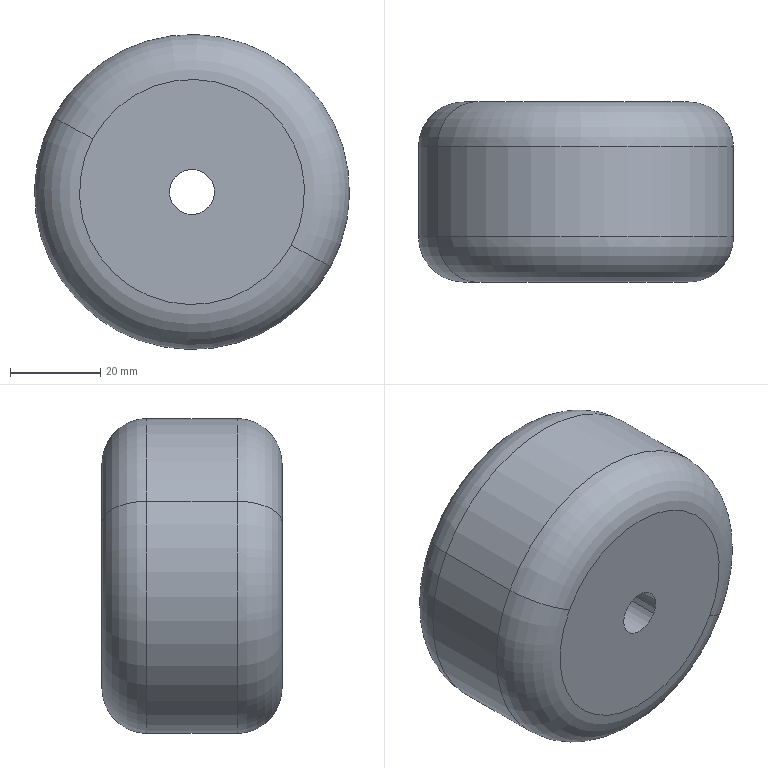Component | SolidWorks | AssemblyVibratoryFeederChassis-1_AssemblyWheel-1_Wheel-1 | 1 solid | 10 faces | box 70 x 40 x 70 mm | volume 141960 mm3 | torus 4 | cylinder 4 | plane 2 | commonest cylinder face diameters 10 x2 70 x2
build123d program:
from build123d import *

# Parameters (mm, degrees)
SKETCH1_R      = 35
SKETCH1_R_2    = 5
EXTRUDE1_DEPTH = 40
FILLET1_R      = 10


with BuildPart() as part:
    # Sketch1 → Extrude1 (new body)
    with BuildSketch(Plane.XY):
        Circle(SKETCH1_R)
        Circle(SKETCH1_R_2, mode=Mode.SUBTRACT)
    extrude(amount=-EXTRUDE1_DEPTH)

    # Fillet1
    fillet1_edges = [part.edges().sort_by_distance(p)[0] for p in [
        (-35, 0, 0),
        (-35, 0, -40),
    ]]
    fillet(fillet1_edges, radius=FILLET1_R)


solid = part.part

# Placed as in the assembly
solid = solid.moved(Location((-277.449, -301.176, -142.722), (90, 0, 0)))
STEP:
#1=COLOUR_RGB('',0.7922,0.8196,0.9333);
#2=FILL_AREA_STYLE_COLOUR('',#1);
#3=FILL_AREA_STYLE('',(#2));
#4=SURFACE_STYLE_FILL_AREA(#3);
#5=SURFACE_SIDE_STYLE('',(#4));
#6=SURFACE_STYLE_USAGE(.BOTH.,#5);
#7=PRESENTATION_STYLE_ASSIGNMENT((#6));
#8=CARTESIAN_POINT('',(-12.137,-11.464,-4.966));
#9=VERTEX_POINT('',#8);
#10=CARTESIAN_POINT('',(-9.71,-11.464,-6.272));
#11=VERTEX_POINT('',#10);
#12=CARTESIAN_POINT('',(-10.923,-11.464,-5.619));
#13=DIRECTION('',(0.,1.,-0.));
#14=DIRECTION('',(0.8806,0.,-0.4738));
#15=AXIS2_PLACEMENT_3D('',#12,#13,#14);
#16=CIRCLE('',#15,1.378);
#17=EDGE_CURVE('',#9,#11,#16,.T.);
#18=ORIENTED_EDGE('',*,*,#17,.F.);
#19=CARTESIAN_POINT('',(-11.79,-11.857,-5.153));
#20=VERTEX_POINT('',#19);
#21=CARTESIAN_POINT('',(-11.79,-11.464,-5.153));
#22=DIRECTION('',(0.4738,0.,0.8806));
#23=DIRECTION('',(0.8806,0.,-0.4738));
#24=AXIS2_PLACEMENT_3D('',#21,#22,#23);
#25=CIRCLE('',#24,0.3937);
#26=EDGE_CURVE('',#9,#20,#25,.T.);
#27=ORIENTED_EDGE('',*,*,#26,.T.);
#28=CARTESIAN_POINT('',(-10.056,-11.857,-6.085));
#29=VERTEX_POINT('',#28);
#30=CARTESIAN_POINT('',(-10.923,-11.857,-5.619));
#31=DIRECTION('',(-0.,-1.,0.));
#32=DIRECTION('',(0.8806,0.,-0.4738));
#33=AXIS2_PLACEMENT_3D('',#30,#31,#32);
#34=CIRCLE('',#33,0.9843);
#35=EDGE_CURVE('',#29,#20,#34,.T.);
#36=ORIENTED_EDGE('',*,*,#35,.F.);
#37=CARTESIAN_POINT('',(-10.056,-11.464,-6.085));
#38=DIRECTION('',(-0.4738,-0.,-0.8806));
#39=DIRECTION('',(-0.8806,0.,0.4738));
#40=AXIS2_PLACEMENT_3D('',#37,#38,#39);
#41=CIRCLE('',#40,0.3937);
#42=EDGE_CURVE('',#11,#29,#41,.T.);
#43=ORIENTED_EDGE('',*,*,#42,.F.);
#44=EDGE_LOOP('',(#18,#27,#36,#43));
#45=FACE_OUTER_BOUND('',#44,.T.);
#46=CARTESIAN_POINT('',(-10.923,-11.464,-5.619));
#47=DIRECTION('',(-0.,-1.,0.));
#48=DIRECTION('',(0.8806,-0.,-0.4738));
#49=AXIS2_PLACEMENT_3D('',#46,#47,#48);
#50=TOROIDAL_SURFACE('',#49,0.9843,0.3937);
#51=ADVANCED_FACE('',(#45),#50,.T.);
#52=CARTESIAN_POINT('',(-11.79,-10.283,-5.153));
#53=VERTEX_POINT('',#52);
#54=CARTESIAN_POINT('',(-10.056,-10.283,-6.085));
#55=VERTEX_POINT('',#54);
#56=CARTESIAN_POINT('',(-10.923,-10.283,-5.619));
#57=DIRECTION('',(0.,1.,-0.));
#58=DIRECTION('',(0.8806,0.,-0.4738));
#59=AXIS2_PLACEMENT_3D('',#56,#57,#58);
#60=CIRCLE('',#59,0.9843);
#61=EDGE_CURVE('',#53,#55,#60,.T.);
#62=ORIENTED_EDGE('',*,*,#61,.F.);
#63=CARTESIAN_POINT('',(-12.137,-10.676,-4.966));
#64=VERTEX_POINT('',#63);
#65=CARTESIAN_POINT('',(-11.79,-10.676,-5.153));
#66=DIRECTION('',(0.4738,0.,0.8806));
#67=DIRECTION('',(0.8806,0.,-0.4738));
#68=AXIS2_PLACEMENT_3D('',#65,#66,#67);
#69=CIRCLE('',#68,0.3937);
#70=EDGE_CURVE('',#53,#64,#69,.T.);
#71=ORIENTED_EDGE('',*,*,#70,.T.);
#72=CARTESIAN_POINT('',(-9.71,-10.676,-6.272));
#73=VERTEX_POINT('',#72);
#74=CARTESIAN_POINT('',(-10.923,-10.676,-5.619));
#75=DIRECTION('',(-0.,-1.,0.));
#76=DIRECTION('',(0.8806,0.,-0.4738));
#77=AXIS2_PLACEMENT_3D('',#74,#75,#76);
#78=CIRCLE('',#77,1.378);
#79=EDGE_CURVE('',#73,#64,#78,.T.);
#80=ORIENTED_EDGE('',*,*,#79,.F.);
#81=CARTESIAN_POINT('',(-10.056,-10.676,-6.085));
#82=DIRECTION('',(-0.4738,-0.,-0.8806));
#83=DIRECTION('',(-0.8806,0.,0.4738));
#84=AXIS2_PLACEMENT_3D('',#81,#82,#83);
#85=CIRCLE('',#84,0.3937);
#86=EDGE_CURVE('',#55,#73,#85,.T.);
#87=ORIENTED_EDGE('',*,*,#86,.F.);
#88=EDGE_LOOP('',(#62,#71,#80,#87));
#89=FACE_OUTER_BOUND('',#88,.T.);
#90=CARTESIAN_POINT('',(-10.923,-10.676,-5.619));
#91=DIRECTION('',(-0.,-1.,0.));
#92=DIRECTION('',(0.8806,-0.,-0.4738));
#93=AXIS2_PLACEMENT_3D('',#90,#91,#92);
#94=TOROIDAL_SURFACE('',#93,0.9843,0.3937);
#95=ADVANCED_FACE('',(#89),#94,.T.);
#96=CARTESIAN_POINT('',(-11.097,-10.283,-5.526));
#97=VERTEX_POINT('',#96);
#98=CARTESIAN_POINT('',(-10.75,-10.283,-5.712));
#99=VERTEX_POINT('',#98);
#100=CARTESIAN_POINT('',(-10.923,-10.283,-5.619));
#101=DIRECTION('',(-0.,-1.,0.));
#102=DIRECTION('',(0.8806,0.,-0.4738));
#103=AXIS2_PLACEMENT_3D('',#100,#101,#102);
#104=CIRCLE('',#103,0.1969);
#105=EDGE_CURVE('',#97,#99,#104,.T.);
#106=ORIENTED_EDGE('',*,*,#105,.F.);
#107=CARTESIAN_POINT('',(-11.097,-11.857,-5.526));
#108=VERTEX_POINT('',#107);
#109=CARTESIAN_POINT('',(-11.097,-10.283,-5.526));
#110=DIRECTION('',(-0.,-1.,0.));
#111=VECTOR('',#110,39.37);
#112=LINE('',#109,#111);
#113=EDGE_CURVE('',#97,#108,#112,.T.);
#114=ORIENTED_EDGE('',*,*,#113,.T.);
#115=CARTESIAN_POINT('',(-10.75,-11.857,-5.712));
#116=VERTEX_POINT('',#115);
#117=CARTESIAN_POINT('',(-10.923,-11.857,-5.619));
#118=DIRECTION('',(-0.,-1.,0.));
#119=DIRECTION('',(0.8806,0.,-0.4738));
#120=AXIS2_PLACEMENT_3D('',#117,#118,#119);
#121=CIRCLE('',#120,0.1969);
#122=EDGE_CURVE('',#108,#116,#121,.T.);
#123=ORIENTED_EDGE('',*,*,#122,.T.);
#124=CARTESIAN_POINT('',(-10.75,-10.283,-5.712));
#125=DIRECTION('',(-0.,-1.,0.));
#126=VECTOR('',#125,39.37);
#127=LINE('',#124,#126);
#128=EDGE_CURVE('',#99,#116,#127,.T.);
#129=ORIENTED_EDGE('',*,*,#128,.F.);
#130=EDGE_LOOP('',(#106,#114,#123,#129));
#131=FACE_OUTER_BOUND('',#130,.T.);
#132=CARTESIAN_POINT('',(-10.923,-10.283,-5.619));
#133=DIRECTION('',(-0.,-1.,0.));
#134=DIRECTION('',(0.8806,0.,-0.4738));
#135=AXIS2_PLACEMENT_3D('',#132,#133,#134);
#136=CYLINDRICAL_SURFACE('',#135,0.1969);
#137=ADVANCED_FACE('',(#131),#136,.F.);
#138=ORIENTED_EDGE('',*,*,#79,.T.);
#139=CARTESIAN_POINT('',(-12.137,-10.283,-4.966));
#140=DIRECTION('',(-0.,-1.,0.));
#141=VECTOR('',#140,39.37);
#142=LINE('',#139,#141);
#143=EDGE_CURVE('',#64,#9,#142,.T.);
#144=ORIENTED_EDGE('',*,*,#143,.T.);
#145=ORIENTED_EDGE('',*,*,#17,.T.);
#146=CARTESIAN_POINT('',(-9.71,-10.283,-6.272));
#147=DIRECTION('',(-0.,-1.,0.));
#148=VECTOR('',#147,39.37);
#149=LINE('',#146,#148);
#150=EDGE_CURVE('',#73,#11,#149,.T.);
#151=ORIENTED_EDGE('',*,*,#150,.F.);
#152=EDGE_LOOP('',(#138,#144,#145,#151));
#153=FACE_OUTER_BOUND('',#152,.T.);
#154=CARTESIAN_POINT('',(-10.923,-10.283,-5.619));
#155=DIRECTION('',(-0.,-1.,0.));
#156=DIRECTION('',(0.8806,0.,-0.4738));
#157=AXIS2_PLACEMENT_3D('',#154,#155,#156);
#158=CYLINDRICAL_SURFACE('',#157,1.378);
#159=ADVANCED_FACE('',(#153),#158,.T.);
#160=ORIENTED_EDGE('',*,*,#143,.F.);
#161=CARTESIAN_POINT('',(-10.923,-10.676,-5.619));
#162=DIRECTION('',(-0.,-1.,0.));
#163=DIRECTION('',(0.8806,0.,-0.4738));
#164=AXIS2_PLACEMENT_3D('',#161,#162,#163);
#165=CIRCLE('',#164,1.378);
#166=EDGE_CURVE('',#64,#73,#165,.T.);
#167=ORIENTED_EDGE('',*,*,#166,.T.);
#168=ORIENTED_EDGE('',*,*,#150,.T.);
#169=CARTESIAN_POINT('',(-10.923,-11.464,-5.619));
#170=DIRECTION('',(0.,1.,-0.));
#171=DIRECTION('',(0.8806,0.,-0.4738));
#172=AXIS2_PLACEMENT_3D('',#169,#170,#171);
#173=CIRCLE('',#172,1.378);
#174=EDGE_CURVE('',#11,#9,#173,.T.);
#175=ORIENTED_EDGE('',*,*,#174,.T.);
#176=EDGE_LOOP('',(#160,#167,#168,#175));
#177=FACE_OUTER_BOUND('',#176,.T.);
#178=CARTESIAN_POINT('',(-10.923,-10.283,-5.619));
#179=DIRECTION('',(-0.,-1.,0.));
#180=DIRECTION('',(0.8806,0.,-0.4738));
#181=AXIS2_PLACEMENT_3D('',#178,#179,#180);
#182=CYLINDRICAL_SURFACE('',#181,1.378);
#183=ADVANCED_FACE('',(#177),#182,.T.);
#184=CARTESIAN_POINT('',(-10.923,-10.283,-5.619));
#185=DIRECTION('',(0.,1.,-0.));
#186=DIRECTION('',(0.8806,0.,-0.4738));
#187=AXIS2_PLACEMENT_3D('',#184,#185,#186);
#188=CIRCLE('',#187,0.9843);
#189=EDGE_CURVE('',#55,#53,#188,.T.);
#190=ORIENTED_EDGE('',*,*,#189,.T.);
#191=ORIENTED_EDGE('',*,*,#61,.T.);
#192=EDGE_LOOP('',(#190,#191));
#193=FACE_OUTER_BOUND('',#192,.T.);
#194=CARTESIAN_POINT('',(-10.923,-10.283,-5.619));
#195=DIRECTION('',(-0.,-1.,0.));
#196=DIRECTION('',(0.8806,0.,-0.4738));
#197=AXIS2_PLACEMENT_3D('',#194,#195,#196);
#198=CIRCLE('',#197,0.1969);
#199=EDGE_CURVE('',#99,#97,#198,.T.);
#200=ORIENTED_EDGE('',*,*,#199,.T.);
#201=ORIENTED_EDGE('',*,*,#105,.T.);
#202=EDGE_LOOP('',(#200,#201));
#203=FACE_BOUND('',#202,.T.);
#204=CARTESIAN_POINT('',(-10.923,-10.283,-5.619));
#205=DIRECTION('',(-0.,-1.,0.));
#206=DIRECTION('',(0.8806,-0.,-0.4738));
#207=AXIS2_PLACEMENT_3D('',#204,#205,#206);
#208=PLANE('',#207);
#209=ADVANCED_FACE('',(#193,#203),#208,.F.);
#210=ORIENTED_EDGE('',*,*,#35,.T.);
#211=CARTESIAN_POINT('',(-10.923,-11.857,-5.619));
#212=DIRECTION('',(-0.,-1.,0.));
#213=DIRECTION('',(0.8806,0.,-0.4738));
#214=AXIS2_PLACEMENT_3D('',#211,#212,#213);
#215=CIRCLE('',#214,0.9843);
#216=EDGE_CURVE('',#20,#29,#215,.T.);
#217=ORIENTED_EDGE('',*,*,#216,.T.);
#218=EDGE_LOOP('',(#210,#217));
#219=FACE_OUTER_BOUND('',#218,.T.);
#220=CARTESIAN_POINT('',(-10.923,-11.857,-5.619));
#221=DIRECTION('',(-0.,-1.,0.));
#222=DIRECTION('',(0.8806,0.,-0.4738));
#223=AXIS2_PLACEMENT_3D('',#220,#221,#222);
#224=CIRCLE('',#223,0.1969);
#225=EDGE_CURVE('',#116,#108,#224,.T.);
#226=ORIENTED_EDGE('',*,*,#225,.F.);
#227=ORIENTED_EDGE('',*,*,#122,.F.);
#228=EDGE_LOOP('',(#226,#227));
#229=FACE_BOUND('',#228,.T.);
#230=CARTESIAN_POINT('',(-10.923,-11.857,-5.619));
#231=DIRECTION('',(-0.,-1.,0.));
#232=DIRECTION('',(0.8806,-0.,-0.4738));
#233=AXIS2_PLACEMENT_3D('',#230,#231,#232);
#234=PLANE('',#233);
#235=ADVANCED_FACE('',(#219,#229),#234,.T.);
#236=ORIENTED_EDGE('',*,*,#113,.F.);
#237=ORIENTED_EDGE('',*,*,#199,.F.);
#238=ORIENTED_EDGE('',*,*,#128,.T.);
#239=ORIENTED_EDGE('',*,*,#225,.T.);
#240=EDGE_LOOP('',(#236,#237,#238,#239));
#241=FACE_OUTER_BOUND('',#240,.T.);
#242=CARTESIAN_POINT('',(-10.923,-10.283,-5.619));
#243=DIRECTION('',(-0.,-1.,0.));
#244=DIRECTION('',(0.8806,0.,-0.4738));
#245=AXIS2_PLACEMENT_3D('',#242,#243,#244);
#246=CYLINDRICAL_SURFACE('',#245,0.1969);
#247=ADVANCED_FACE('',(#241),#246,.F.);
#248=ORIENTED_EDGE('',*,*,#70,.F.);
#249=ORIENTED_EDGE('',*,*,#189,.F.);
#250=ORIENTED_EDGE('',*,*,#86,.T.);
#251=ORIENTED_EDGE('',*,*,#166,.F.);
#252=EDGE_LOOP('',(#248,#249,#250,#251));
#253=FACE_OUTER_BOUND('',#252,.T.);
#254=CARTESIAN_POINT('',(-10.923,-10.676,-5.619));
#255=DIRECTION('',(-0.,-1.,0.));
#256=DIRECTION('',(0.8806,-0.,-0.4738));
#257=AXIS2_PLACEMENT_3D('',#254,#255,#256);
#258=TOROIDAL_SURFACE('',#257,0.9843,0.3937);
#259=ADVANCED_FACE('',(#253),#258,.T.);
#260=ORIENTED_EDGE('',*,*,#26,.F.);
#261=ORIENTED_EDGE('',*,*,#174,.F.);
#262=ORIENTED_EDGE('',*,*,#42,.T.);
#263=ORIENTED_EDGE('',*,*,#216,.F.);
#264=EDGE_LOOP('',(#260,#261,#262,#263));
#265=FACE_OUTER_BOUND('',#264,.T.);
#266=CARTESIAN_POINT('',(-10.923,-11.464,-5.619));
#267=DIRECTION('',(-0.,-1.,0.));
#268=DIRECTION('',(0.8806,-0.,-0.4738));
#269=AXIS2_PLACEMENT_3D('',#266,#267,#268);
#270=TOROIDAL_SURFACE('',#269,0.9843,0.3937);
#271=ADVANCED_FACE('',(#265),#270,.T.);
#272=CLOSED_SHELL('',(#51,#95,#137,#159,#183,#209,#235,#247,#259,#271));
#273=MANIFOLD_SOLID_BREP('',#272);
#274=STYLED_ITEM('',(#7),#273);
#275=(LENGTH_UNIT()NAMED_UNIT(*)SI_UNIT($,.METRE.));
#276=LENGTH_MEASURE_WITH_UNIT(LENGTH_MEASURE(0.0254),#275);
#277=DIMENSIONAL_EXPONENTS(1.,0.,0.,0.,0.,0.,0.);
#278=(CONVERSION_BASED_UNIT('',#276)LENGTH_UNIT()NAMED_UNIT(#277));
#279=UNCERTAINTY_MEASURE_WITH_UNIT(LENGTH_MEASURE(0.00001),#278,'','');
#280=(NAMED_UNIT(*)PLANE_ANGLE_UNIT()SI_UNIT($,.RADIAN.));
#281=(NAMED_UNIT(*)SI_UNIT($,.STERADIAN.)SOLID_ANGLE_UNIT());
#282=(GEOMETRIC_REPRESENTATION_CONTEXT(3)GLOBAL_UNCERTAINTY_ASSIGNED_CONTEXT((#279))GLOBAL_UNIT_ASSIGNED_CONTEXT((#278,#280,#281))REPRESENTATION_CONTEXT('',''));
#283=MECHANICAL_DESIGN_GEOMETRIC_PRESENTATION_REPRESENTATION('',(#274),#282);
#284=PRESENTATION_LAYER_ASSIGNMENT('','',(#274));
#285=CARTESIAN_POINT('',(0.,0.,0.));
#286=DIRECTION('',(0.,0.,1.));
#287=DIRECTION('',(1.,0.,0.));
#288=AXIS2_PLACEMENT_3D('',#285,#286,#287);
#289=(LENGTH_UNIT()NAMED_UNIT(*)SI_UNIT($,.METRE.));
#290=LENGTH_MEASURE_WITH_UNIT(LENGTH_MEASURE(0.0254),#289);
#291=DIMENSIONAL_EXPONENTS(1.,0.,0.,0.,0.,0.,0.);
#292=(CONVERSION_BASED_UNIT('',#290)LENGTH_UNIT()NAMED_UNIT(#291));
#293=UNCERTAINTY_MEASURE_WITH_UNIT(LENGTH_MEASURE(0.00001),#292,'','');
#294=(NAMED_UNIT(*)PLANE_ANGLE_UNIT()SI_UNIT($,.RADIAN.));
#295=(NAMED_UNIT(*)SI_UNIT($,.STERADIAN.)SOLID_ANGLE_UNIT());
#296=(GEOMETRIC_REPRESENTATION_CONTEXT(3)GLOBAL_UNCERTAINTY_ASSIGNED_CONTEXT((#293))GLOBAL_UNIT_ASSIGNED_CONTEXT((#292,#294,#295))REPRESENTATION_CONTEXT('',''));
#297=ADVANCED_BREP_SHAPE_REPRESENTATION('',(#273,#288),#296);